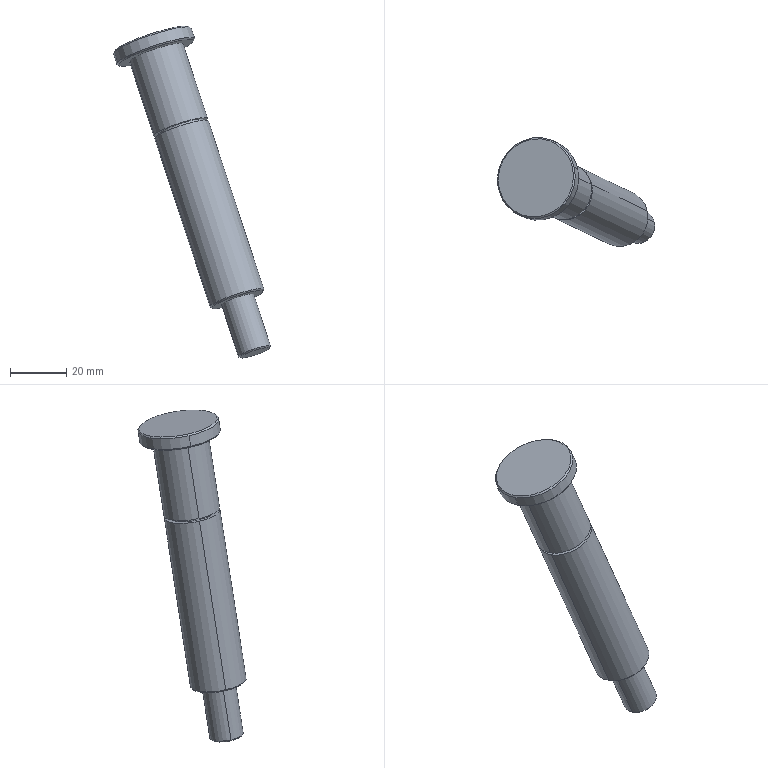Component | SolidWorks | FilmPressingSoilCoveringMechanism2Reverse-2_AttachedSoilDiskAssembly2-1_LargeAttachedSoilDiskAxis-1 | 1 solid | 24 faces | box 55.69 x 38.39 x 117.55 mm | volume 34659 mm3 | cylinder 10 | cone 8 | plane 6 | commonest cylinder face diameters 20 x4 29 x2 17 x2 12 x2
build123d program:
from build123d import *

# Parameters (mm, degrees)
SKETCH1_R           = 14.5
BOSS_EXTRUDE1_DEPTH = 5
SKETCH3_R           = 10
BOSS_EXTRUDE2_DEPTH = 93
SKETCH4_R           = 6
BOSS_EXTRUDE3_DEPTH = 20
SKETCH5_W           = 3
SKETCH5_H           = 1
CHAMFER1_SIZE       = 0.5
CHAMFER2_SIZE       = 0.5


with BuildPart() as part:
    # Sketch1 → Boss-Extrude1 (new body)
    with BuildSketch(Plane.XY):
        Circle(SKETCH1_R)
    extrude(amount=BOSS_EXTRUDE1_DEPTH)

    # Sketch3 → Boss-Extrude2 (add)
    with BuildSketch(Plane.XY.offset(5)):
        with Locations(Location((0, 0, 0), (0, 0, 180))):
            Circle(SKETCH3_R)
    extrude(amount=BOSS_EXTRUDE2_DEPTH)

    # Sketch4 → Boss-Extrude3 (add)
    with BuildSketch(Plane.XY.offset(98)):
        Circle(SKETCH4_R)
    extrude(amount=BOSS_EXTRUDE3_DEPTH)

    # Sketch5 → Cut-Revolve1 (revolve, cut)
    with BuildSketch(Plane(origin=(0, 0, 0), x_dir=(1, 0, 0), z_dir=(0, 1, 0))):
        with Locations((-10, -33.5)):
            Rectangle(SKETCH5_W, SKETCH5_H)
    revolve(axis=Axis((0, 0, 0), (0, 0, 1)), mode=Mode.SUBTRACT)

    # Chamfer1
    chamfer1_edges = [part.edges().sort_by_distance(p)[0] for p in [
        (-6, 0, 118),
        (10, 0, 98),
    ]]
    chamfer(chamfer1_edges, length=CHAMFER1_SIZE)

    # Chamfer2
    chamfer2_edges = [part.edges().sort_by_distance(p)[0] for p in [
        (-14.5, 0, 0),
        (-14.5, 0, 5),
    ]]
    chamfer(chamfer2_edges, length=CHAMFER2_SIZE)


solid = part.part

# Placed as in the assembly
solid = solid.moved(Location((-1935.799, -296.223, 2641.267), (171.174, 18.019, 29.782)))
STEP:
#1=CARTESIAN_POINT('',(-76.724,-11.808,103.841));
#2=VERTEX_POINT('',#1);
#3=CARTESIAN_POINT('',(-75.701,-11.517,104.133));
#4=VERTEX_POINT('',#3);
#5=CARTESIAN_POINT('',(-76.213,-11.662,103.987));
#6=DIRECTION('',(-0.3093,0.1459,0.9397));
#7=DIRECTION('',(0.9277,0.2635,0.2645));
#8=AXIS2_PLACEMENT_3D('',#5,#6,#7);
#9=CIRCLE('',#8,0.5512);
#10=EDGE_CURVE('',#2,#4,#9,.T.);
#11=ORIENTED_EDGE('',*,*,#10,.F.);
#12=CARTESIAN_POINT('',(-76.736,-11.816,103.817));
#13=VERTEX_POINT('',#12);
#14=CARTESIAN_POINT('',(-76.736,-11.816,103.817));
#15=DIRECTION('',(-0.4373,-0.2895,-0.8515));
#16=VECTOR('',#15,39.37);
#17=LINE('',#14,#16);
#18=EDGE_CURVE('',#2,#13,#17,.T.);
#19=ORIENTED_EDGE('',*,*,#18,.T.);
#20=CARTESIAN_POINT('',(-75.677,-11.515,104.119));
#21=VERTEX_POINT('',#20);
#22=CARTESIAN_POINT('',(-76.206,-11.665,103.968));
#23=DIRECTION('',(0.3093,-0.1459,-0.9397));
#24=DIRECTION('',(0.9277,0.2635,0.2645));
#25=AXIS2_PLACEMENT_3D('',#22,#23,#24);
#26=CIRCLE('',#25,0.5709);
#27=EDGE_CURVE('',#21,#13,#26,.T.);
#28=ORIENTED_EDGE('',*,*,#27,.F.);
#29=CARTESIAN_POINT('',(-75.677,-11.515,104.119));
#30=DIRECTION('',(0.8747,0.08312,-0.4774));
#31=VECTOR('',#30,39.37);
#32=LINE('',#29,#31);
#33=EDGE_CURVE('',#4,#21,#32,.T.);
#34=ORIENTED_EDGE('',*,*,#33,.F.);
#35=EDGE_LOOP('',(#11,#19,#28,#34));
#36=FACE_OUTER_BOUND('',#35,.T.);
#37=CARTESIAN_POINT('',(-76.206,-11.665,103.968));
#38=DIRECTION('',(0.3093,-0.1459,-0.9397));
#39=DIRECTION('',(0.9277,0.2635,0.2645));
#40=AXIS2_PLACEMENT_3D('',#37,#38,#39);
#41=CONICAL_SURFACE('',#40,0.5709,0.7854);
#42=ADVANCED_FACE('',(#36),#41,.T.);
#43=CARTESIAN_POINT('',(-75.64,-11.546,103.948));
#44=VERTEX_POINT('',#43);
#45=CARTESIAN_POINT('',(-76.663,-11.836,103.656));
#46=VERTEX_POINT('',#45);
#47=CARTESIAN_POINT('',(-76.152,-11.691,103.802));
#48=DIRECTION('',(0.3093,-0.1459,-0.9397));
#49=DIRECTION('',(0.9277,0.2635,0.2645));
#50=AXIS2_PLACEMENT_3D('',#47,#48,#49);
#51=CIRCLE('',#50,0.5512);
#52=EDGE_CURVE('',#44,#46,#51,.T.);
#53=ORIENTED_EDGE('',*,*,#52,.F.);
#54=CARTESIAN_POINT('',(-75.628,-11.538,103.971));
#55=VERTEX_POINT('',#54);
#56=CARTESIAN_POINT('',(-75.64,-11.546,103.948));
#57=DIRECTION('',(0.4373,0.2895,0.8515));
#58=VECTOR('',#57,39.37);
#59=LINE('',#56,#58);
#60=EDGE_CURVE('',#44,#55,#59,.T.);
#61=ORIENTED_EDGE('',*,*,#60,.T.);
#62=CARTESIAN_POINT('',(-76.687,-11.839,103.669));
#63=VERTEX_POINT('',#62);
#64=CARTESIAN_POINT('',(-76.158,-11.688,103.82));
#65=DIRECTION('',(-0.3093,0.1459,0.9397));
#66=DIRECTION('',(0.9277,0.2635,0.2645));
#67=AXIS2_PLACEMENT_3D('',#64,#65,#66);
#68=CIRCLE('',#67,0.5709);
#69=EDGE_CURVE('',#63,#55,#68,.T.);
#70=ORIENTED_EDGE('',*,*,#69,.F.);
#71=CARTESIAN_POINT('',(-76.663,-11.836,103.656));
#72=DIRECTION('',(-0.8747,-0.08312,0.4774));
#73=VECTOR('',#72,39.37);
#74=LINE('',#71,#73);
#75=EDGE_CURVE('',#46,#63,#74,.T.);
#76=ORIENTED_EDGE('',*,*,#75,.F.);
#77=EDGE_LOOP('',(#53,#61,#70,#76));
#78=FACE_OUTER_BOUND('',#77,.T.);
#79=CARTESIAN_POINT('',(-76.152,-11.691,103.802));
#80=DIRECTION('',(-0.3093,0.1459,0.9397));
#81=DIRECTION('',(-0.9277,-0.2635,-0.2645));
#82=AXIS2_PLACEMENT_3D('',#79,#80,#81);
#83=CONICAL_SURFACE('',#82,0.5512,0.7854);
#84=ADVANCED_FACE('',(#78),#83,.T.);
#85=CARTESIAN_POINT('',(-74.575,-12.283,99.679));
#86=VERTEX_POINT('',#85);
#87=CARTESIAN_POINT('',(-74.976,-12.397,99.564));
#88=VERTEX_POINT('',#87);
#89=CARTESIAN_POINT('',(-74.775,-12.34,99.621));
#90=DIRECTION('',(0.3093,-0.1459,-0.9397));
#91=DIRECTION('',(0.9277,0.2635,0.2645));
#92=AXIS2_PLACEMENT_3D('',#89,#90,#91);
#93=CIRCLE('',#92,0.2165);
#94=EDGE_CURVE('',#86,#88,#93,.T.);
#95=ORIENTED_EDGE('',*,*,#94,.F.);
#96=CARTESIAN_POINT('',(-74.562,-12.275,99.702));
#97=VERTEX_POINT('',#96);
#98=CARTESIAN_POINT('',(-74.575,-12.283,99.679));
#99=DIRECTION('',(0.4373,0.2895,0.8515));
#100=VECTOR('',#99,39.37);
#101=LINE('',#98,#100);
#102=EDGE_CURVE('',#86,#97,#101,.T.);
#103=ORIENTED_EDGE('',*,*,#102,.T.);
#104=CARTESIAN_POINT('',(-75.001,-12.4,99.577));
#105=VERTEX_POINT('',#104);
#106=CARTESIAN_POINT('',(-74.782,-12.337,99.64));
#107=DIRECTION('',(-0.3093,0.1459,0.9397));
#108=DIRECTION('',(0.9277,0.2635,0.2645));
#109=AXIS2_PLACEMENT_3D('',#106,#107,#108);
#110=CIRCLE('',#109,0.2362);
#111=EDGE_CURVE('',#105,#97,#110,.T.);
#112=ORIENTED_EDGE('',*,*,#111,.F.);
#113=CARTESIAN_POINT('',(-74.976,-12.397,99.564));
#114=DIRECTION('',(-0.8747,-0.08312,0.4774));
#115=VECTOR('',#114,39.37);
#116=LINE('',#113,#115);
#117=EDGE_CURVE('',#88,#105,#116,.T.);
#118=ORIENTED_EDGE('',*,*,#117,.F.);
#119=EDGE_LOOP('',(#95,#103,#112,#118));
#120=FACE_OUTER_BOUND('',#119,.T.);
#121=CARTESIAN_POINT('',(-74.775,-12.34,99.621));
#122=DIRECTION('',(-0.3093,0.1459,0.9397));
#123=DIRECTION('',(-0.9277,-0.2635,-0.2645));
#124=AXIS2_PLACEMENT_3D('',#121,#122,#123);
#125=CONICAL_SURFACE('',#124,0.2165,0.7854);
#126=ADVANCED_FACE('',(#120),#125,.T.);
#127=CARTESIAN_POINT('',(-74.672,-12.127,100.46));
#128=VERTEX_POINT('',#127);
#129=CARTESIAN_POINT('',(-75.366,-12.324,100.262));
#130=VERTEX_POINT('',#129);
#131=CARTESIAN_POINT('',(-75.019,-12.225,100.361));
#132=DIRECTION('',(0.3093,-0.1459,-0.9397));
#133=DIRECTION('',(0.9277,0.2635,0.2645));
#134=AXIS2_PLACEMENT_3D('',#131,#132,#133);
#135=CIRCLE('',#134,0.374);
#136=EDGE_CURVE('',#128,#130,#135,.T.);
#137=ORIENTED_EDGE('',*,*,#136,.F.);
#138=CARTESIAN_POINT('',(-74.66,-12.119,100.484));
#139=VERTEX_POINT('',#138);
#140=CARTESIAN_POINT('',(-74.672,-12.127,100.46));
#141=DIRECTION('',(0.4373,0.2895,0.8515));
#142=VECTOR('',#141,39.37);
#143=LINE('',#140,#142);
#144=EDGE_CURVE('',#128,#139,#143,.T.);
#145=ORIENTED_EDGE('',*,*,#144,.T.);
#146=CARTESIAN_POINT('',(-75.39,-12.326,100.276));
#147=VERTEX_POINT('',#146);
#148=CARTESIAN_POINT('',(-75.025,-12.222,100.38));
#149=DIRECTION('',(-0.3093,0.1459,0.9397));
#150=DIRECTION('',(0.9277,0.2635,0.2645));
#151=AXIS2_PLACEMENT_3D('',#148,#149,#150);
#152=CIRCLE('',#151,0.3937);
#153=EDGE_CURVE('',#147,#139,#152,.T.);
#154=ORIENTED_EDGE('',*,*,#153,.F.);
#155=CARTESIAN_POINT('',(-75.366,-12.324,100.262));
#156=DIRECTION('',(-0.8747,-0.08312,0.4774));
#157=VECTOR('',#156,39.37);
#158=LINE('',#155,#157);
#159=EDGE_CURVE('',#130,#147,#158,.T.);
#160=ORIENTED_EDGE('',*,*,#159,.F.);
#161=EDGE_LOOP('',(#137,#145,#154,#160));
#162=FACE_OUTER_BOUND('',#161,.T.);
#163=CARTESIAN_POINT('',(-75.019,-12.225,100.361));
#164=DIRECTION('',(-0.3093,0.1459,0.9397));
#165=DIRECTION('',(-0.9277,-0.2635,-0.2645));
#166=AXIS2_PLACEMENT_3D('',#163,#164,#165);
#167=CONICAL_SURFACE('',#166,0.374,0.7854);
#168=ADVANCED_FACE('',(#162),#167,.T.);
#169=CARTESIAN_POINT('',(-76.176,-11.956,102.662));
#170=VERTEX_POINT('',#169);
#171=CARTESIAN_POINT('',(-75.445,-11.748,102.87));
#172=VERTEX_POINT('',#171);
#173=CARTESIAN_POINT('',(-75.811,-11.852,102.766));
#174=DIRECTION('',(-0.3093,0.1459,0.9397));
#175=DIRECTION('',(-0.9277,-0.2635,-0.2645));
#176=AXIS2_PLACEMENT_3D('',#173,#174,#175);
#177=CIRCLE('',#176,0.3937);
#178=EDGE_CURVE('',#170,#172,#177,.T.);
#179=ORIENTED_EDGE('',*,*,#178,.T.);
#180=CARTESIAN_POINT('',(-75.786,-11.587,103.906));
#181=VERTEX_POINT('',#180);
#182=CARTESIAN_POINT('',(-74.654,-12.122,100.465));
#183=DIRECTION('',(-0.3093,0.1459,0.9397));
#184=VECTOR('',#183,39.37);
#185=LINE('',#182,#184);
#186=EDGE_CURVE('',#172,#181,#185,.T.);
#187=ORIENTED_EDGE('',*,*,#186,.T.);
#188=CARTESIAN_POINT('',(-76.517,-11.795,103.698));
#189=VERTEX_POINT('',#188);
#190=CARTESIAN_POINT('',(-76.152,-11.691,103.802));
#191=DIRECTION('',(0.3093,-0.1459,-0.9397));
#192=DIRECTION('',(0.9277,0.2635,0.2645));
#193=AXIS2_PLACEMENT_3D('',#190,#191,#192);
#194=CIRCLE('',#193,0.3937);
#195=EDGE_CURVE('',#181,#189,#194,.T.);
#196=ORIENTED_EDGE('',*,*,#195,.T.);
#197=CARTESIAN_POINT('',(-75.384,-12.329,100.257));
#198=DIRECTION('',(-0.3093,0.1459,0.9397));
#199=VECTOR('',#198,39.37);
#200=LINE('',#197,#199);
#201=EDGE_CURVE('',#170,#189,#200,.T.);
#202=ORIENTED_EDGE('',*,*,#201,.F.);
#203=EDGE_LOOP('',(#179,#187,#196,#202));
#204=FACE_OUTER_BOUND('',#203,.T.);
#205=CARTESIAN_POINT('',(-75.019,-12.225,100.361));
#206=DIRECTION('',(-0.3093,0.1459,0.9397));
#207=DIRECTION('',(-0.9277,-0.2635,-0.2645));
#208=AXIS2_PLACEMENT_3D('',#205,#206,#207);
#209=CYLINDRICAL_SURFACE('',#208,0.3937);
#210=ADVANCED_FACE('',(#204),#209,.T.);
#211=ORIENTED_EDGE('',*,*,#69,.T.);
#212=CARTESIAN_POINT('',(-75.622,-11.541,103.953));
#213=DIRECTION('',(-0.3093,0.1459,0.9397));
#214=VECTOR('',#213,39.37);
#215=LINE('',#212,#214);
#216=EDGE_CURVE('',#55,#21,#215,.T.);
#217=ORIENTED_EDGE('',*,*,#216,.T.);
#218=ORIENTED_EDGE('',*,*,#27,.T.);
#219=CARTESIAN_POINT('',(-76.681,-11.841,103.651));
#220=DIRECTION('',(-0.3093,0.1459,0.9397));
#221=VECTOR('',#220,39.37);
#222=LINE('',#219,#221);
#223=EDGE_CURVE('',#63,#13,#222,.T.);
#224=ORIENTED_EDGE('',*,*,#223,.F.);
#225=EDGE_LOOP('',(#211,#217,#218,#224));
#226=FACE_OUTER_BOUND('',#225,.T.);
#227=CARTESIAN_POINT('',(-76.152,-11.691,103.802));
#228=DIRECTION('',(-0.3093,0.1459,0.9397));
#229=DIRECTION('',(-0.9277,-0.2635,-0.2645));
#230=AXIS2_PLACEMENT_3D('',#227,#228,#229);
#231=CYLINDRICAL_SURFACE('',#230,0.5709);
#232=ADVANCED_FACE('',(#226),#231,.T.);
#233=CARTESIAN_POINT('',(-76.109,-11.946,102.641));
#234=VERTEX_POINT('',#233);
#235=CARTESIAN_POINT('',(-75.488,-11.769,102.818));
#236=VERTEX_POINT('',#235);
#237=CARTESIAN_POINT('',(-75.798,-11.858,102.729));
#238=DIRECTION('',(-0.3093,0.1459,0.9397));
#239=DIRECTION('',(-0.9277,-0.2635,-0.2645));
#240=AXIS2_PLACEMENT_3D('',#237,#238,#239);
#241=CIRCLE('',#240,0.3346);
#242=EDGE_CURVE('',#234,#236,#241,.T.);
#243=ORIENTED_EDGE('',*,*,#242,.T.);
#244=CARTESIAN_POINT('',(-75.5,-11.764,102.855));
#245=VERTEX_POINT('',#244);
#246=CARTESIAN_POINT('',(-75.902,-11.574,104.075));
#247=DIRECTION('',(-0.3093,0.1459,0.9397));
#248=VECTOR('',#247,39.37);
#249=LINE('',#246,#248);
#250=EDGE_CURVE('',#236,#245,#249,.T.);
#251=ORIENTED_EDGE('',*,*,#250,.T.);
#252=CARTESIAN_POINT('',(-76.121,-11.94,102.678));
#253=VERTEX_POINT('',#252);
#254=CARTESIAN_POINT('',(-75.811,-11.852,102.766));
#255=DIRECTION('',(-0.3093,0.1459,0.9397));
#256=DIRECTION('',(-0.9277,-0.2635,-0.2645));
#257=AXIS2_PLACEMENT_3D('',#254,#255,#256);
#258=CIRCLE('',#257,0.3346);
#259=EDGE_CURVE('',#253,#245,#258,.T.);
#260=ORIENTED_EDGE('',*,*,#259,.F.);
#261=CARTESIAN_POINT('',(-76.523,-11.75,103.898));
#262=DIRECTION('',(-0.3093,0.1459,0.9397));
#263=VECTOR('',#262,39.37);
#264=LINE('',#261,#263);
#265=EDGE_CURVE('',#234,#253,#264,.T.);
#266=ORIENTED_EDGE('',*,*,#265,.F.);
#267=EDGE_LOOP('',(#243,#251,#260,#266));
#268=FACE_OUTER_BOUND('',#267,.T.);
#269=CARTESIAN_POINT('',(-76.213,-11.662,103.987));
#270=DIRECTION('',(-0.3093,0.1459,0.9397));
#271=DIRECTION('',(-0.9277,-0.2635,-0.2645));
#272=AXIS2_PLACEMENT_3D('',#269,#270,#271);
#273=CYLINDRICAL_SURFACE('',#272,0.3346);
#274=ADVANCED_FACE('',(#268),#273,.T.);
#275=ORIENTED_EDGE('',*,*,#111,.T.);
#276=CARTESIAN_POINT('',(-74.8,-12.163,100.424));
#277=VERTEX_POINT('',#276);
#278=CARTESIAN_POINT('',(-74.556,-12.278,99.684));
#279=DIRECTION('',(-0.3093,0.1459,0.9397));
#280=VECTOR('',#279,39.37);
#281=LINE('',#278,#280);
#282=EDGE_CURVE('',#97,#277,#281,.T.);
#283=ORIENTED_EDGE('',*,*,#282,.T.);
#284=CARTESIAN_POINT('',(-75.238,-12.288,100.299));
#285=VERTEX_POINT('',#284);
#286=CARTESIAN_POINT('',(-75.019,-12.225,100.361));
#287=DIRECTION('',(0.3093,-0.1459,-0.9397));
#288=DIRECTION('',(0.9277,0.2635,0.2645));
#289=AXIS2_PLACEMENT_3D('',#286,#287,#288);
#290=CIRCLE('',#289,0.2362);
#291=EDGE_CURVE('',#277,#285,#290,.T.);
#292=ORIENTED_EDGE('',*,*,#291,.T.);
#293=CARTESIAN_POINT('',(-74.995,-12.402,99.559));
#294=DIRECTION('',(-0.3093,0.1459,0.9397));
#295=VECTOR('',#294,39.37);
#296=LINE('',#293,#295);
#297=EDGE_CURVE('',#105,#285,#296,.T.);
#298=ORIENTED_EDGE('',*,*,#297,.F.);
#299=EDGE_LOOP('',(#275,#283,#292,#298));
#300=FACE_OUTER_BOUND('',#299,.T.);
#301=CARTESIAN_POINT('',(-74.775,-12.34,99.621));
#302=DIRECTION('',(-0.3093,0.1459,0.9397));
#303=DIRECTION('',(-0.9277,-0.2635,-0.2645));
#304=AXIS2_PLACEMENT_3D('',#301,#302,#303);
#305=CYLINDRICAL_SURFACE('',#304,0.2362);
#306=ADVANCED_FACE('',(#300),#305,.T.);
#307=ORIENTED_EDGE('',*,*,#153,.T.);
#308=CARTESIAN_POINT('',(-75.433,-11.754,102.833));
#309=VERTEX_POINT('',#308);
#310=CARTESIAN_POINT('',(-74.654,-12.122,100.465));
#311=DIRECTION('',(-0.3093,0.1459,0.9397));
#312=VECTOR('',#311,39.37);
#313=LINE('',#310,#312);
#314=EDGE_CURVE('',#139,#309,#313,.T.);
#315=ORIENTED_EDGE('',*,*,#314,.T.);
#316=CARTESIAN_POINT('',(-76.164,-11.961,102.625));
#317=VERTEX_POINT('',#316);
#318=CARTESIAN_POINT('',(-75.798,-11.858,102.729));
#319=DIRECTION('',(0.3093,-0.1459,-0.9397));
#320=DIRECTION('',(0.9277,0.2635,0.2645));
#321=AXIS2_PLACEMENT_3D('',#318,#319,#320);
#322=CIRCLE('',#321,0.3937);
#323=EDGE_CURVE('',#309,#317,#322,.T.);
#324=ORIENTED_EDGE('',*,*,#323,.T.);
#325=CARTESIAN_POINT('',(-75.384,-12.329,100.257));
#326=DIRECTION('',(-0.3093,0.1459,0.9397));
#327=VECTOR('',#326,39.37);
#328=LINE('',#325,#327);
#329=EDGE_CURVE('',#147,#317,#328,.T.);
#330=ORIENTED_EDGE('',*,*,#329,.F.);
#331=EDGE_LOOP('',(#307,#315,#324,#330));
#332=FACE_OUTER_BOUND('',#331,.T.);
#333=CARTESIAN_POINT('',(-75.019,-12.225,100.361));
#334=DIRECTION('',(-0.3093,0.1459,0.9397));
#335=DIRECTION('',(-0.9277,-0.2635,-0.2645));
#336=AXIS2_PLACEMENT_3D('',#333,#334,#335);
#337=CYLINDRICAL_SURFACE('',#336,0.3937);
#338=ADVANCED_FACE('',(#332),#337,.T.);
#339=ORIENTED_EDGE('',*,*,#314,.F.);
#340=CARTESIAN_POINT('',(-75.025,-12.222,100.38));
#341=DIRECTION('',(-0.3093,0.1459,0.9397));
#342=DIRECTION('',(0.9277,0.2635,0.2645));
#343=AXIS2_PLACEMENT_3D('',#340,#341,#342);
#344=CIRCLE('',#343,0.3937);
#345=EDGE_CURVE('',#139,#147,#344,.T.);
#346=ORIENTED_EDGE('',*,*,#345,.T.);
#347=ORIENTED_EDGE('',*,*,#329,.T.);
#348=CARTESIAN_POINT('',(-75.798,-11.858,102.729));
#349=DIRECTION('',(0.3093,-0.1459,-0.9397));
#350=DIRECTION('',(0.9277,0.2635,0.2645));
#351=AXIS2_PLACEMENT_3D('',#348,#349,#350);
#352=CIRCLE('',#351,0.3937);
#353=EDGE_CURVE('',#317,#309,#352,.T.);
#354=ORIENTED_EDGE('',*,*,#353,.T.);
#355=EDGE_LOOP('',(#339,#346,#347,#354));
#356=FACE_OUTER_BOUND('',#355,.T.);
#357=CARTESIAN_POINT('',(-75.019,-12.225,100.361));
#358=DIRECTION('',(-0.3093,0.1459,0.9397));
#359=DIRECTION('',(-0.9277,-0.2635,-0.2645));
#360=AXIS2_PLACEMENT_3D('',#357,#358,#359);
#361=CYLINDRICAL_SURFACE('',#360,0.3937);
#362=ADVANCED_FACE('',(#356),#361,.T.);
#363=CARTESIAN_POINT('',(-75.019,-12.225,100.361));
#364=DIRECTION('',(0.3093,-0.1459,-0.9397));
#365=DIRECTION('',(0.9277,0.2635,0.2645));
#366=AXIS2_PLACEMENT_3D('',#363,#364,#365);
#367=CIRCLE('',#366,0.374);
#368=EDGE_CURVE('',#130,#128,#367,.T.);
#369=ORIENTED_EDGE('',*,*,#368,.T.);
#370=ORIENTED_EDGE('',*,*,#136,.T.);
#371=EDGE_LOOP('',(#369,#370));
#372=FACE_OUTER_BOUND('',#371,.T.);
#373=CARTESIAN_POINT('',(-75.019,-12.225,100.361));
#374=DIRECTION('',(0.3093,-0.1459,-0.9397));
#375=DIRECTION('',(0.9277,0.2635,0.2645));
#376=AXIS2_PLACEMENT_3D('',#373,#374,#375);
#377=CIRCLE('',#376,0.2362);
#378=EDGE_CURVE('',#285,#277,#377,.T.);
#379=ORIENTED_EDGE('',*,*,#378,.F.);
#380=ORIENTED_EDGE('',*,*,#291,.F.);
#381=EDGE_LOOP('',(#379,#380));
#382=FACE_BOUND('',#381,.T.);
#383=CARTESIAN_POINT('',(-75.019,-12.225,100.361));
#384=DIRECTION('',(0.3093,-0.1459,-0.9397));
#385=DIRECTION('',(0.9277,0.2635,0.2645));
#386=AXIS2_PLACEMENT_3D('',#383,#384,#385);
#387=PLANE('',#386);
#388=ADVANCED_FACE('',(#372,#382),#387,.T.);
#389=ORIENTED_EDGE('',*,*,#282,.F.);
#390=CARTESIAN_POINT('',(-74.782,-12.337,99.64));
#391=DIRECTION('',(-0.3093,0.1459,0.9397));
#392=DIRECTION('',(0.9277,0.2635,0.2645));
#393=AXIS2_PLACEMENT_3D('',#390,#391,#392);
#394=CIRCLE('',#393,0.2362);
#395=EDGE_CURVE('',#97,#105,#394,.T.);
#396=ORIENTED_EDGE('',*,*,#395,.T.);
#397=ORIENTED_EDGE('',*,*,#297,.T.);
#398=ORIENTED_EDGE('',*,*,#378,.T.);
#399=EDGE_LOOP('',(#389,#396,#397,#398));
#400=FACE_OUTER_BOUND('',#399,.T.);
#401=CARTESIAN_POINT('',(-74.775,-12.34,99.621));
#402=DIRECTION('',(-0.3093,0.1459,0.9397));
#403=DIRECTION('',(-0.9277,-0.2635,-0.2645));
#404=AXIS2_PLACEMENT_3D('',#401,#402,#403);
#405=CYLINDRICAL_SURFACE('',#404,0.2362);
#406=ADVANCED_FACE('',(#400),#405,.T.);
#407=CARTESIAN_POINT('',(-74.775,-12.34,99.621));
#408=DIRECTION('',(0.3093,-0.1459,-0.9397));
#409=DIRECTION('',(0.9277,0.2635,0.2645));
#410=AXIS2_PLACEMENT_3D('',#407,#408,#409);
#411=CIRCLE('',#410,0.2165);
#412=EDGE_CURVE('',#88,#86,#411,.T.);
#413=ORIENTED_EDGE('',*,*,#412,.T.);
#414=ORIENTED_EDGE('',*,*,#94,.T.);
#415=EDGE_LOOP('',(#413,#414));
#416=FACE_OUTER_BOUND('',#415,.T.);
#417=CARTESIAN_POINT('',(-74.775,-12.34,99.621));
#418=DIRECTION('',(0.3093,-0.1459,-0.9397));
#419=DIRECTION('',(0.9277,0.2635,0.2645));
#420=AXIS2_PLACEMENT_3D('',#417,#418,#419);
#421=PLANE('',#420);
#422=ADVANCED_FACE('',(#416),#421,.T.);
#423=ORIENTED_EDGE('',*,*,#242,.F.);
#424=CARTESIAN_POINT('',(-75.798,-11.858,102.729));
#425=DIRECTION('',(-0.3093,0.1459,0.9397));
#426=DIRECTION('',(-0.9277,-0.2635,-0.2645));
#427=AXIS2_PLACEMENT_3D('',#424,#425,#426);
#428=CIRCLE('',#427,0.3346);
#429=EDGE_CURVE('',#236,#234,#428,.T.);
#430=ORIENTED_EDGE('',*,*,#429,.F.);
#431=EDGE_LOOP('',(#423,#430));
#432=FACE_BOUND('',#431,.T.);
#433=ORIENTED_EDGE('',*,*,#353,.F.);
#434=ORIENTED_EDGE('',*,*,#323,.F.);
#435=EDGE_LOOP('',(#433,#434));
#436=FACE_OUTER_BOUND('',#435,.T.);
#437=CARTESIAN_POINT('',(-76.219,-11.977,102.609));
#438=DIRECTION('',(0.3093,-0.1459,-0.9397));
#439=DIRECTION('',(0.9277,0.2635,0.2645));
#440=AXIS2_PLACEMENT_3D('',#437,#438,#439);
#441=PLANE('',#440);
#442=ADVANCED_FACE('',(#432,#436),#441,.F.);
#443=ORIENTED_EDGE('',*,*,#259,.T.);
#444=CARTESIAN_POINT('',(-75.811,-11.852,102.766));
#445=DIRECTION('',(-0.3093,0.1459,0.9397));
#446=DIRECTION('',(-0.9277,-0.2635,-0.2645));
#447=AXIS2_PLACEMENT_3D('',#444,#445,#446);
#448=CIRCLE('',#447,0.3346);
#449=EDGE_CURVE('',#245,#253,#448,.T.);
#450=ORIENTED_EDGE('',*,*,#449,.T.);
#451=EDGE_LOOP('',(#443,#450));
#452=FACE_BOUND('',#451,.T.);
#453=ORIENTED_EDGE('',*,*,#178,.F.);
#454=CARTESIAN_POINT('',(-75.811,-11.852,102.766));
#455=DIRECTION('',(-0.3093,0.1459,0.9397));
#456=DIRECTION('',(-0.9277,-0.2635,-0.2645));
#457=AXIS2_PLACEMENT_3D('',#454,#455,#456);
#458=CIRCLE('',#457,0.3937);
#459=EDGE_CURVE('',#172,#170,#458,.T.);
#460=ORIENTED_EDGE('',*,*,#459,.F.);
#461=EDGE_LOOP('',(#453,#460));
#462=FACE_OUTER_BOUND('',#461,.T.);
#463=CARTESIAN_POINT('',(-76.231,-11.971,102.646));
#464=DIRECTION('',(-0.3093,0.1459,0.9397));
#465=DIRECTION('',(-0.9277,-0.2635,-0.2645));
#466=AXIS2_PLACEMENT_3D('',#463,#464,#465);
#467=PLANE('',#466);
#468=ADVANCED_FACE('',(#452,#462),#467,.F.);
#469=ORIENTED_EDGE('',*,*,#250,.F.);
#470=ORIENTED_EDGE('',*,*,#429,.T.);
#471=ORIENTED_EDGE('',*,*,#265,.T.);
#472=ORIENTED_EDGE('',*,*,#449,.F.);
#473=EDGE_LOOP('',(#469,#470,#471,#472));
#474=FACE_OUTER_BOUND('',#473,.T.);
#475=CARTESIAN_POINT('',(-76.213,-11.662,103.987));
#476=DIRECTION('',(-0.3093,0.1459,0.9397));
#477=DIRECTION('',(-0.9277,-0.2635,-0.2645));
#478=AXIS2_PLACEMENT_3D('',#475,#476,#477);
#479=CYLINDRICAL_SURFACE('',#478,0.3346);
#480=ADVANCED_FACE('',(#474),#479,.T.);
#481=CARTESIAN_POINT('',(-76.213,-11.662,103.987));
#482=DIRECTION('',(-0.3093,0.1459,0.9397));
#483=DIRECTION('',(0.9277,0.2635,0.2645));
#484=AXIS2_PLACEMENT_3D('',#481,#482,#483);
#485=CIRCLE('',#484,0.5512);
#486=EDGE_CURVE('',#4,#2,#485,.T.);
#487=ORIENTED_EDGE('',*,*,#486,.T.);
#488=ORIENTED_EDGE('',*,*,#10,.T.);
#489=EDGE_LOOP('',(#487,#488));
#490=FACE_OUTER_BOUND('',#489,.T.);
#491=CARTESIAN_POINT('',(-76.213,-11.662,103.987));
#492=DIRECTION('',(0.3093,-0.1459,-0.9397));
#493=DIRECTION('',(0.9277,0.2635,0.2645));
#494=AXIS2_PLACEMENT_3D('',#491,#492,#493);
#495=PLANE('',#494);
#496=ADVANCED_FACE('',(#490),#495,.F.);
#497=ORIENTED_EDGE('',*,*,#216,.F.);
#498=CARTESIAN_POINT('',(-76.158,-11.688,103.82));
#499=DIRECTION('',(-0.3093,0.1459,0.9397));
#500=DIRECTION('',(0.9277,0.2635,0.2645));
#501=AXIS2_PLACEMENT_3D('',#498,#499,#500);
#502=CIRCLE('',#501,0.5709);
#503=EDGE_CURVE('',#55,#63,#502,.T.);
#504=ORIENTED_EDGE('',*,*,#503,.T.);
#505=ORIENTED_EDGE('',*,*,#223,.T.);
#506=CARTESIAN_POINT('',(-76.206,-11.665,103.968));
#507=DIRECTION('',(0.3093,-0.1459,-0.9397));
#508=DIRECTION('',(0.9277,0.2635,0.2645));
#509=AXIS2_PLACEMENT_3D('',#506,#507,#508);
#510=CIRCLE('',#509,0.5709);
#511=EDGE_CURVE('',#13,#21,#510,.T.);
#512=ORIENTED_EDGE('',*,*,#511,.T.);
#513=EDGE_LOOP('',(#497,#504,#505,#512));
#514=FACE_OUTER_BOUND('',#513,.T.);
#515=CARTESIAN_POINT('',(-76.152,-11.691,103.802));
#516=DIRECTION('',(-0.3093,0.1459,0.9397));
#517=DIRECTION('',(-0.9277,-0.2635,-0.2645));
#518=AXIS2_PLACEMENT_3D('',#515,#516,#517);
#519=CYLINDRICAL_SURFACE('',#518,0.5709);
#520=ADVANCED_FACE('',(#514),#519,.T.);
#521=CARTESIAN_POINT('',(-76.152,-11.691,103.802));
#522=DIRECTION('',(0.3093,-0.1459,-0.9397));
#523=DIRECTION('',(0.9277,0.2635,0.2645));
#524=AXIS2_PLACEMENT_3D('',#521,#522,#523);
#525=CIRCLE('',#524,0.5512);
#526=EDGE_CURVE('',#46,#44,#525,.T.);
#527=ORIENTED_EDGE('',*,*,#526,.T.);
#528=ORIENTED_EDGE('',*,*,#52,.T.);
#529=EDGE_LOOP('',(#527,#528));
#530=FACE_OUTER_BOUND('',#529,.T.);
#531=CARTESIAN_POINT('',(-76.152,-11.691,103.802));
#532=DIRECTION('',(0.3093,-0.1459,-0.9397));
#533=DIRECTION('',(0.9277,0.2635,0.2645));
#534=AXIS2_PLACEMENT_3D('',#531,#532,#533);
#535=CIRCLE('',#534,0.3937);
#536=EDGE_CURVE('',#189,#181,#535,.T.);
#537=ORIENTED_EDGE('',*,*,#536,.F.);
#538=ORIENTED_EDGE('',*,*,#195,.F.);
#539=EDGE_LOOP('',(#537,#538));
#540=FACE_BOUND('',#539,.T.);
#541=CARTESIAN_POINT('',(-76.152,-11.691,103.802));
#542=DIRECTION('',(0.3093,-0.1459,-0.9397));
#543=DIRECTION('',(0.9277,0.2635,0.2645));
#544=AXIS2_PLACEMENT_3D('',#541,#542,#543);
#545=PLANE('',#544);
#546=ADVANCED_FACE('',(#530,#540),#545,.T.);
#547=ORIENTED_EDGE('',*,*,#186,.F.);
#548=ORIENTED_EDGE('',*,*,#459,.T.);
#549=ORIENTED_EDGE('',*,*,#201,.T.);
#550=ORIENTED_EDGE('',*,*,#536,.T.);
#551=EDGE_LOOP('',(#547,#548,#549,#550));
#552=FACE_OUTER_BOUND('',#551,.T.);
#553=CARTESIAN_POINT('',(-75.019,-12.225,100.361));
#554=DIRECTION('',(-0.3093,0.1459,0.9397));
#555=DIRECTION('',(-0.9277,-0.2635,-0.2645));
#556=AXIS2_PLACEMENT_3D('',#553,#554,#555);
#557=CYLINDRICAL_SURFACE('',#556,0.3937);
#558=ADVANCED_FACE('',(#552),#557,.T.);
#559=ORIENTED_EDGE('',*,*,#144,.F.);
#560=ORIENTED_EDGE('',*,*,#368,.F.);
#561=ORIENTED_EDGE('',*,*,#159,.T.);
#562=ORIENTED_EDGE('',*,*,#345,.F.);
#563=EDGE_LOOP('',(#559,#560,#561,#562));
#564=FACE_OUTER_BOUND('',#563,.T.);
#565=CARTESIAN_POINT('',(-75.019,-12.225,100.361));
#566=DIRECTION('',(-0.3093,0.1459,0.9397));
#567=DIRECTION('',(-0.9277,-0.2635,-0.2645));
#568=AXIS2_PLACEMENT_3D('',#565,#566,#567);
#569=CONICAL_SURFACE('',#568,0.374,0.7854);
#570=ADVANCED_FACE('',(#564),#569,.T.);
#571=ORIENTED_EDGE('',*,*,#102,.F.);
#572=ORIENTED_EDGE('',*,*,#412,.F.);
#573=ORIENTED_EDGE('',*,*,#117,.T.);
#574=ORIENTED_EDGE('',*,*,#395,.F.);
#575=EDGE_LOOP('',(#571,#572,#573,#574));
#576=FACE_OUTER_BOUND('',#575,.T.);
#577=CARTESIAN_POINT('',(-74.775,-12.34,99.621));
#578=DIRECTION('',(-0.3093,0.1459,0.9397));
#579=DIRECTION('',(-0.9277,-0.2635,-0.2645));
#580=AXIS2_PLACEMENT_3D('',#577,#578,#579);
#581=CONICAL_SURFACE('',#580,0.2165,0.7854);
#582=ADVANCED_FACE('',(#576),#581,.T.);
#583=ORIENTED_EDGE('',*,*,#60,.F.);
#584=ORIENTED_EDGE('',*,*,#526,.F.);
#585=ORIENTED_EDGE('',*,*,#75,.T.);
#586=ORIENTED_EDGE('',*,*,#503,.F.);
#587=EDGE_LOOP('',(#583,#584,#585,#586));
#588=FACE_OUTER_BOUND('',#587,.T.);
#589=CARTESIAN_POINT('',(-76.152,-11.691,103.802));
#590=DIRECTION('',(-0.3093,0.1459,0.9397));
#591=DIRECTION('',(-0.9277,-0.2635,-0.2645));
#592=AXIS2_PLACEMENT_3D('',#589,#590,#591);
#593=CONICAL_SURFACE('',#592,0.5512,0.7854);
#594=ADVANCED_FACE('',(#588),#593,.T.);
#595=ORIENTED_EDGE('',*,*,#18,.F.);
#596=ORIENTED_EDGE('',*,*,#486,.F.);
#597=ORIENTED_EDGE('',*,*,#33,.T.);
#598=ORIENTED_EDGE('',*,*,#511,.F.);
#599=EDGE_LOOP('',(#595,#596,#597,#598));
#600=FACE_OUTER_BOUND('',#599,.T.);
#601=CARTESIAN_POINT('',(-76.206,-11.665,103.968));
#602=DIRECTION('',(0.3093,-0.1459,-0.9397));
#603=DIRECTION('',(0.9277,0.2635,0.2645));
#604=AXIS2_PLACEMENT_3D('',#601,#602,#603);
#605=CONICAL_SURFACE('',#604,0.5709,0.7854);
#606=ADVANCED_FACE('',(#600),#605,.T.);
#607=CLOSED_SHELL('',(#42,#84,#126,#168,#210,#232,#274,#306,#338,#362,#388,#406,#422,#442,#468,#480,#496,#520,#546,#558,#570,#582,#594,#606));
#608=MANIFOLD_SOLID_BREP('',#607);
#609=CARTESIAN_POINT('',(0.,0.,0.));
#610=DIRECTION('',(0.,0.,1.));
#611=DIRECTION('',(1.,0.,0.));
#612=AXIS2_PLACEMENT_3D('',#609,#610,#611);
#613=(LENGTH_UNIT()NAMED_UNIT(*)SI_UNIT($,.METRE.));
#614=LENGTH_MEASURE_WITH_UNIT(LENGTH_MEASURE(0.0254),#613);
#615=DIMENSIONAL_EXPONENTS(1.,0.,0.,0.,0.,0.,0.);
#616=(CONVERSION_BASED_UNIT('',#614)LENGTH_UNIT()NAMED_UNIT(#615));
#617=UNCERTAINTY_MEASURE_WITH_UNIT(LENGTH_MEASURE(0.00001),#616,'','');
#618=(NAMED_UNIT(*)PLANE_ANGLE_UNIT()SI_UNIT($,.RADIAN.));
#619=(NAMED_UNIT(*)SI_UNIT($,.STERADIAN.)SOLID_ANGLE_UNIT());
#620=(GEOMETRIC_REPRESENTATION_CONTEXT(3)GLOBAL_UNCERTAINTY_ASSIGNED_CONTEXT((#617))GLOBAL_UNIT_ASSIGNED_CONTEXT((#616,#618,#619))REPRESENTATION_CONTEXT('',''));
#621=ADVANCED_BREP_SHAPE_REPRESENTATION('',(#608,#612),#620);
#622=COLOUR_RGB('',0.7922,0.8196,0.9333);
#623=FILL_AREA_STYLE_COLOUR('',#622);
#624=FILL_AREA_STYLE('',(#623));
#625=SURFACE_STYLE_FILL_AREA(#624);
#626=SURFACE_SIDE_STYLE('',(#625));
#627=SURFACE_STYLE_USAGE(.BOTH.,#626);
#628=PRESENTATION_STYLE_ASSIGNMENT((#627));
#629=STYLED_ITEM('',(#628),#608);
#630=(LENGTH_UNIT()NAMED_UNIT(*)SI_UNIT($,.METRE.));
#631=LENGTH_MEASURE_WITH_UNIT(LENGTH_MEASURE(0.0254),#630);
#632=DIMENSIONAL_EXPONENTS(1.,0.,0.,0.,0.,0.,0.);
#633=(CONVERSION_BASED_UNIT('',#631)LENGTH_UNIT()NAMED_UNIT(#632));
#634=UNCERTAINTY_MEASURE_WITH_UNIT(LENGTH_MEASURE(0.00001),#633,'','');
#635=(NAMED_UNIT(*)PLANE_ANGLE_UNIT()SI_UNIT($,.RADIAN.));
#636=(NAMED_UNIT(*)SI_UNIT($,.STERADIAN.)SOLID_ANGLE_UNIT());
#637=(GEOMETRIC_REPRESENTATION_CONTEXT(3)GLOBAL_UNCERTAINTY_ASSIGNED_CONTEXT((#634))GLOBAL_UNIT_ASSIGNED_CONTEXT((#633,#635,#636))REPRESENTATION_CONTEXT('',''));
#638=MECHANICAL_DESIGN_GEOMETRIC_PRESENTATION_REPRESENTATION('',(#629),#637);
#639=PRESENTATION_LAYER_ASSIGNMENT('','',(#629));